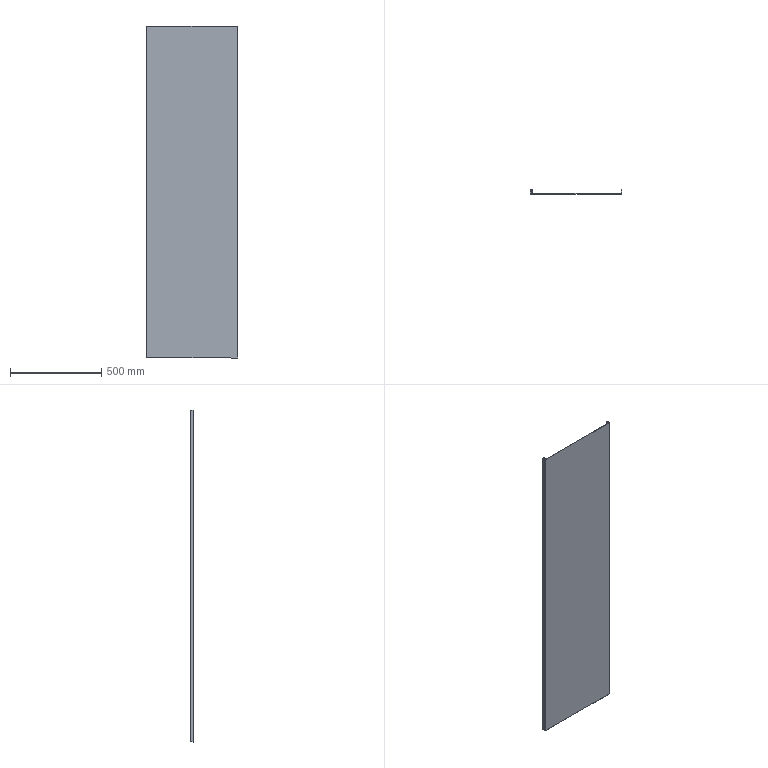Component | SolidWorks | SidePlate-1 | 1 solid | 38 faces | box 500 x 20 x 1820 mm | volume 1504835 mm3 | plane 30 | cylinder 8 | commonest cylinder face diameters 5 x2 2 x2 4.473 x2 1.473 x2
STEP:
#1=COLOUR_RGB('',0.7922,0.8196,0.9333);
#2=FILL_AREA_STYLE_COLOUR('',#1);
#3=FILL_AREA_STYLE('',(#2));
#4=SURFACE_STYLE_FILL_AREA(#3);
#5=SURFACE_SIDE_STYLE('',(#4));
#6=SURFACE_STYLE_USAGE(.BOTH.,#5);
#7=PRESENTATION_STYLE_ASSIGNMENT((#6));
#8=CARTESIAN_POINT('',(0.2466,-9.272,66.594));
#9=VERTEX_POINT('',#8);
#10=CARTESIAN_POINT('',(0.029,-9.272,66.594));
#11=VERTEX_POINT('',#10);
#12=CARTESIAN_POINT('',(9.783,-9.272,66.594));
#13=DIRECTION('',(-1.,-0.,0.));
#14=VECTOR('',#13,39.37);
#15=LINE('',#12,#14);
#16=EDGE_CURVE('',#9,#11,#15,.T.);
#17=ORIENTED_EDGE('',*,*,#16,.F.);
#18=CARTESIAN_POINT('',(0.2466,-9.213,66.594));
#19=VERTEX_POINT('',#18);
#20=CARTESIAN_POINT('',(0.2466,-9.272,66.594));
#21=DIRECTION('',(0.,1.,0.));
#22=VECTOR('',#21,39.37);
#23=LINE('',#20,#22);
#24=EDGE_CURVE('',#9,#19,#23,.T.);
#25=ORIENTED_EDGE('',*,*,#24,.T.);
#26=CARTESIAN_POINT('',(0.029,-9.213,66.594));
#27=VERTEX_POINT('',#26);
#28=CARTESIAN_POINT('',(0.,-9.213,66.594));
#29=DIRECTION('',(-1.,-0.,0.));
#30=VECTOR('',#29,39.37);
#31=LINE('',#28,#30);
#32=EDGE_CURVE('',#19,#27,#31,.T.);
#33=ORIENTED_EDGE('',*,*,#32,.T.);
#34=CARTESIAN_POINT('',(0.029,-9.272,66.594));
#35=DIRECTION('',(-0.,1.,0.));
#36=VECTOR('',#35,39.37);
#37=LINE('',#34,#36);
#38=EDGE_CURVE('',#11,#27,#37,.T.);
#39=ORIENTED_EDGE('',*,*,#38,.F.);
#40=EDGE_LOOP('',(#17,#25,#33,#39));
#41=FACE_OUTER_BOUND('',#40,.T.);
#42=CARTESIAN_POINT('',(0.,-9.213,66.594));
#43=DIRECTION('',(0.,-0.,1.));
#44=DIRECTION('',(-1.,0.,0.));
#45=AXIS2_PLACEMENT_3D('',#42,#43,#44);
#46=PLANE('',#45);
#47=ADVANCED_FACE('',(#41),#46,.T.);
#48=ORIENTED_EDGE('',*,*,#32,.F.);
#49=CARTESIAN_POINT('',(0.2466,-9.213,-5.059));
#50=VERTEX_POINT('',#49);
#51=CARTESIAN_POINT('',(0.2466,-9.213,66.594));
#52=DIRECTION('',(-0.,0.,-1.));
#53=VECTOR('',#52,39.37);
#54=LINE('',#51,#53);
#55=EDGE_CURVE('',#19,#50,#54,.T.);
#56=ORIENTED_EDGE('',*,*,#55,.T.);
#57=CARTESIAN_POINT('',(0.029,-9.213,-5.059));
#58=VERTEX_POINT('',#57);
#59=CARTESIAN_POINT('',(0.3346,-9.213,-5.059));
#60=DIRECTION('',(1.,0.,-0.));
#61=VECTOR('',#60,39.37);
#62=LINE('',#59,#61);
#63=EDGE_CURVE('',#58,#50,#62,.T.);
#64=ORIENTED_EDGE('',*,*,#63,.F.);
#65=CARTESIAN_POINT('',(0.029,-9.213,30.768));
#66=DIRECTION('',(0.,-0.,1.));
#67=VECTOR('',#66,39.37);
#68=LINE('',#65,#67);
#69=EDGE_CURVE('',#58,#27,#68,.T.);
#70=ORIENTED_EDGE('',*,*,#69,.T.);
#71=EDGE_LOOP('',(#48,#56,#64,#70));
#72=FACE_OUTER_BOUND('',#71,.T.);
#73=CARTESIAN_POINT('',(9.783,-9.213,30.768));
#74=DIRECTION('',(-0.,1.,0.));
#75=DIRECTION('',(1.,0.,-0.));
#76=AXIS2_PLACEMENT_3D('',#73,#74,#75);
#77=PLANE('',#76);
#78=ADVANCED_FACE('',(#72),#77,.T.);
#79=CARTESIAN_POINT('',(0.2466,-9.272,-5.059));
#80=VERTEX_POINT('',#79);
#81=CARTESIAN_POINT('',(0.2466,-9.272,66.594));
#82=DIRECTION('',(-0.,0.,-1.));
#83=VECTOR('',#82,39.37);
#84=LINE('',#81,#83);
#85=EDGE_CURVE('',#9,#80,#84,.T.);
#86=ORIENTED_EDGE('',*,*,#85,.F.);
#87=ORIENTED_EDGE('',*,*,#16,.T.);
#88=CARTESIAN_POINT('',(0.029,-9.272,-5.059));
#89=VERTEX_POINT('',#88);
#90=CARTESIAN_POINT('',(0.029,-9.272,-5.059));
#91=DIRECTION('',(0.,-0.,1.));
#92=VECTOR('',#91,39.37);
#93=LINE('',#90,#92);
#94=EDGE_CURVE('',#89,#11,#93,.T.);
#95=ORIENTED_EDGE('',*,*,#94,.F.);
#96=CARTESIAN_POINT('',(9.783,-9.272,-5.059));
#97=DIRECTION('',(1.,0.,-0.));
#98=VECTOR('',#97,39.37);
#99=LINE('',#96,#98);
#100=EDGE_CURVE('',#89,#80,#99,.T.);
#101=ORIENTED_EDGE('',*,*,#100,.T.);
#102=EDGE_LOOP('',(#86,#87,#95,#101));
#103=FACE_OUTER_BOUND('',#102,.T.);
#104=CARTESIAN_POINT('',(9.783,-9.272,30.768));
#105=DIRECTION('',(-0.,1.,0.));
#106=DIRECTION('',(1.,0.,-0.));
#107=AXIS2_PLACEMENT_3D('',#104,#105,#106);
#108=PLANE('',#107);
#109=ADVANCED_FACE('',(#103),#108,.F.);
#110=CARTESIAN_POINT('',(0.,-9.301,66.594));
#111=VERTEX_POINT('',#110);
#112=CARTESIAN_POINT('',(0.,-9.902,66.594));
#113=VERTEX_POINT('',#112);
#114=CARTESIAN_POINT('',(0.,-10.,66.594));
#115=DIRECTION('',(0.,-1.,-0.));
#116=VECTOR('',#115,39.37);
#117=LINE('',#114,#116);
#118=EDGE_CURVE('',#111,#113,#117,.T.);
#119=ORIENTED_EDGE('',*,*,#118,.F.);
#120=CARTESIAN_POINT('',(-0.05906,-9.301,66.594));
#121=VERTEX_POINT('',#120);
#122=CARTESIAN_POINT('',(0.,-9.301,66.594));
#123=DIRECTION('',(-1.,-0.,0.));
#124=VECTOR('',#123,39.37);
#125=LINE('',#122,#124);
#126=EDGE_CURVE('',#111,#121,#125,.T.);
#127=ORIENTED_EDGE('',*,*,#126,.T.);
#128=CARTESIAN_POINT('',(-0.05906,-9.902,66.594));
#129=VERTEX_POINT('',#128);
#130=CARTESIAN_POINT('',(-0.05906,-9.213,66.594));
#131=DIRECTION('',(0.,-1.,-0.));
#132=VECTOR('',#131,39.37);
#133=LINE('',#130,#132);
#134=EDGE_CURVE('',#121,#129,#133,.T.);
#135=ORIENTED_EDGE('',*,*,#134,.T.);
#136=CARTESIAN_POINT('',(0.,-9.902,66.594));
#137=DIRECTION('',(-1.,0.,0.));
#138=VECTOR('',#137,39.37);
#139=LINE('',#136,#138);
#140=EDGE_CURVE('',#113,#129,#139,.T.);
#141=ORIENTED_EDGE('',*,*,#140,.F.);
#142=EDGE_LOOP('',(#119,#127,#135,#141));
#143=FACE_OUTER_BOUND('',#142,.T.);
#144=CARTESIAN_POINT('',(-0.05906,-9.213,66.594));
#145=DIRECTION('',(0.,-0.,1.));
#146=DIRECTION('',(-1.,0.,0.));
#147=AXIS2_PLACEMENT_3D('',#144,#145,#146);
#148=PLANE('',#147);
#149=ADVANCED_FACE('',(#143),#148,.T.);
#150=CARTESIAN_POINT('',(-0.05906,-9.301,-5.059));
#151=VERTEX_POINT('',#150);
#152=CARTESIAN_POINT('',(-0.05906,-9.301,66.594));
#153=DIRECTION('',(-0.,0.,-1.));
#154=VECTOR('',#153,39.37);
#155=LINE('',#152,#154);
#156=EDGE_CURVE('',#121,#151,#155,.T.);
#157=ORIENTED_EDGE('',*,*,#156,.T.);
#158=CARTESIAN_POINT('',(-0.05906,-9.902,-5.059));
#159=VERTEX_POINT('',#158);
#160=CARTESIAN_POINT('',(-0.05906,-9.941,-5.059));
#161=DIRECTION('',(-0.,1.,0.));
#162=VECTOR('',#161,39.37);
#163=LINE('',#160,#162);
#164=EDGE_CURVE('',#159,#151,#163,.T.);
#165=ORIENTED_EDGE('',*,*,#164,.F.);
#166=CARTESIAN_POINT('',(-0.05906,-9.902,-5.059));
#167=DIRECTION('',(-0.,0.,-1.));
#168=VECTOR('',#167,39.37);
#169=LINE('',#166,#168);
#170=EDGE_CURVE('',#129,#159,#169,.T.);
#171=ORIENTED_EDGE('',*,*,#170,.F.);
#172=ORIENTED_EDGE('',*,*,#134,.F.);
#173=EDGE_LOOP('',(#157,#165,#171,#172));
#174=FACE_OUTER_BOUND('',#173,.T.);
#175=CARTESIAN_POINT('',(-0.05906,-10.,30.768));
#176=DIRECTION('',(1.,0.,-0.));
#177=DIRECTION('',(0.,-1.,-0.));
#178=AXIS2_PLACEMENT_3D('',#175,#176,#177);
#179=PLANE('',#178);
#180=ADVANCED_FACE('',(#174),#179,.F.);
#181=CARTESIAN_POINT('',(0.,-9.902,-5.059));
#182=VERTEX_POINT('',#181);
#183=CARTESIAN_POINT('',(0.,-9.301,-5.059));
#184=VERTEX_POINT('',#183);
#185=CARTESIAN_POINT('',(0.,-10.,-5.059));
#186=DIRECTION('',(-0.,1.,0.));
#187=VECTOR('',#186,39.37);
#188=LINE('',#185,#187);
#189=EDGE_CURVE('',#182,#184,#188,.T.);
#190=ORIENTED_EDGE('',*,*,#189,.T.);
#191=CARTESIAN_POINT('',(0.,-9.301,66.594));
#192=DIRECTION('',(-0.,0.,-1.));
#193=VECTOR('',#192,39.37);
#194=LINE('',#191,#193);
#195=EDGE_CURVE('',#111,#184,#194,.T.);
#196=ORIENTED_EDGE('',*,*,#195,.F.);
#197=ORIENTED_EDGE('',*,*,#118,.T.);
#198=CARTESIAN_POINT('',(0.,-9.902,-5.059));
#199=DIRECTION('',(0.,-0.,1.));
#200=VECTOR('',#199,39.37);
#201=LINE('',#198,#200);
#202=EDGE_CURVE('',#182,#113,#201,.T.);
#203=ORIENTED_EDGE('',*,*,#202,.F.);
#204=EDGE_LOOP('',(#190,#196,#197,#203));
#205=FACE_OUTER_BOUND('',#204,.T.);
#206=CARTESIAN_POINT('',(0.,-10.,30.768));
#207=DIRECTION('',(1.,0.,-0.));
#208=DIRECTION('',(0.,-1.,-0.));
#209=AXIS2_PLACEMENT_3D('',#206,#207,#208);
#210=PLANE('',#209);
#211=ADVANCED_FACE('',(#205),#210,.T.);
#212=CARTESIAN_POINT('',(0.03937,-9.941,66.594));
#213=VERTEX_POINT('',#212);
#214=CARTESIAN_POINT('',(0.03937,-9.941,-5.059));
#215=VERTEX_POINT('',#214);
#216=CARTESIAN_POINT('',(0.03937,-9.941,66.594));
#217=DIRECTION('',(-0.,0.,-1.));
#218=VECTOR('',#217,39.37);
#219=LINE('',#216,#218);
#220=EDGE_CURVE('',#213,#215,#219,.T.);
#221=ORIENTED_EDGE('',*,*,#220,.F.);
#222=CARTESIAN_POINT('',(19.528,-9.941,66.594));
#223=VERTEX_POINT('',#222);
#224=CARTESIAN_POINT('',(19.626,-9.941,66.594));
#225=DIRECTION('',(-1.,0.,0.));
#226=VECTOR('',#225,39.37);
#227=LINE('',#224,#226);
#228=EDGE_CURVE('',#223,#213,#227,.T.);
#229=ORIENTED_EDGE('',*,*,#228,.F.);
#230=CARTESIAN_POINT('',(19.528,-9.941,-5.059));
#231=VERTEX_POINT('',#230);
#232=CARTESIAN_POINT('',(19.528,-9.941,-5.059));
#233=DIRECTION('',(0.,-0.,1.));
#234=VECTOR('',#233,39.37);
#235=LINE('',#232,#234);
#236=EDGE_CURVE('',#231,#223,#235,.T.);
#237=ORIENTED_EDGE('',*,*,#236,.F.);
#238=CARTESIAN_POINT('',(19.626,-9.941,-5.059));
#239=DIRECTION('',(1.,-0.,-0.));
#240=VECTOR('',#239,39.37);
#241=LINE('',#238,#240);
#242=EDGE_CURVE('',#215,#231,#241,.T.);
#243=ORIENTED_EDGE('',*,*,#242,.F.);
#244=EDGE_LOOP('',(#221,#229,#237,#243));
#245=FACE_OUTER_BOUND('',#244,.T.);
#246=CARTESIAN_POINT('',(9.783,-9.941,30.768));
#247=DIRECTION('',(-0.,-1.,-0.));
#248=DIRECTION('',(-1.,0.,0.));
#249=AXIS2_PLACEMENT_3D('',#246,#247,#248);
#250=PLANE('',#249);
#251=ADVANCED_FACE('',(#245),#250,.F.);
#252=CARTESIAN_POINT('',(19.528,-10.,66.594));
#253=VERTEX_POINT('',#252);
#254=CARTESIAN_POINT('',(0.03937,-10.,66.594));
#255=VERTEX_POINT('',#254);
#256=CARTESIAN_POINT('',(19.626,-10.,66.594));
#257=DIRECTION('',(-1.,0.,0.));
#258=VECTOR('',#257,39.37);
#259=LINE('',#256,#258);
#260=EDGE_CURVE('',#253,#255,#259,.T.);
#261=ORIENTED_EDGE('',*,*,#260,.T.);
#262=CARTESIAN_POINT('',(0.03937,-10.,-5.059));
#263=VERTEX_POINT('',#262);
#264=CARTESIAN_POINT('',(0.03937,-10.,66.594));
#265=DIRECTION('',(-0.,0.,-1.));
#266=VECTOR('',#265,39.37);
#267=LINE('',#264,#266);
#268=EDGE_CURVE('',#255,#263,#267,.T.);
#269=ORIENTED_EDGE('',*,*,#268,.T.);
#270=CARTESIAN_POINT('',(19.528,-10.,-5.059));
#271=VERTEX_POINT('',#270);
#272=CARTESIAN_POINT('',(19.626,-10.,-5.059));
#273=DIRECTION('',(1.,-0.,-0.));
#274=VECTOR('',#273,39.37);
#275=LINE('',#272,#274);
#276=EDGE_CURVE('',#263,#271,#275,.T.);
#277=ORIENTED_EDGE('',*,*,#276,.T.);
#278=CARTESIAN_POINT('',(19.528,-10.,-5.059));
#279=DIRECTION('',(0.,-0.,1.));
#280=VECTOR('',#279,39.37);
#281=LINE('',#278,#280);
#282=EDGE_CURVE('',#271,#253,#281,.T.);
#283=ORIENTED_EDGE('',*,*,#282,.T.);
#284=EDGE_LOOP('',(#261,#269,#277,#283));
#285=FACE_OUTER_BOUND('',#284,.T.);
#286=CARTESIAN_POINT('',(9.783,-10.,30.768));
#287=DIRECTION('',(-0.,-1.,-0.));
#288=DIRECTION('',(-1.,0.,0.));
#289=AXIS2_PLACEMENT_3D('',#286,#287,#288);
#290=PLANE('',#289);
#291=ADVANCED_FACE('',(#285),#290,.T.);
#292=ORIENTED_EDGE('',*,*,#228,.T.);
#293=CARTESIAN_POINT('',(0.03937,-9.941,66.594));
#294=DIRECTION('',(-0.,-1.,-0.));
#295=VECTOR('',#294,39.37);
#296=LINE('',#293,#295);
#297=EDGE_CURVE('',#213,#255,#296,.T.);
#298=ORIENTED_EDGE('',*,*,#297,.T.);
#299=ORIENTED_EDGE('',*,*,#260,.F.);
#300=CARTESIAN_POINT('',(19.528,-9.941,66.594));
#301=DIRECTION('',(-0.,-1.,-0.));
#302=VECTOR('',#301,39.37);
#303=LINE('',#300,#302);
#304=EDGE_CURVE('',#223,#253,#303,.T.);
#305=ORIENTED_EDGE('',*,*,#304,.F.);
#306=EDGE_LOOP('',(#292,#298,#299,#305));
#307=FACE_OUTER_BOUND('',#306,.T.);
#308=CARTESIAN_POINT('',(19.626,-9.941,66.594));
#309=DIRECTION('',(0.,-0.,1.));
#310=DIRECTION('',(-1.,0.,0.));
#311=AXIS2_PLACEMENT_3D('',#308,#309,#310);
#312=PLANE('',#311);
#313=ADVANCED_FACE('',(#307),#312,.T.);
#314=CARTESIAN_POINT('',(0.03937,-9.941,-5.059));
#315=DIRECTION('',(-0.,-1.,-0.));
#316=VECTOR('',#315,39.37);
#317=LINE('',#314,#316);
#318=EDGE_CURVE('',#215,#263,#317,.T.);
#319=ORIENTED_EDGE('',*,*,#318,.F.);
#320=ORIENTED_EDGE('',*,*,#242,.T.);
#321=CARTESIAN_POINT('',(19.528,-9.941,-5.059));
#322=DIRECTION('',(-0.,-1.,-0.));
#323=VECTOR('',#322,39.37);
#324=LINE('',#321,#323);
#325=EDGE_CURVE('',#231,#271,#324,.T.);
#326=ORIENTED_EDGE('',*,*,#325,.T.);
#327=ORIENTED_EDGE('',*,*,#276,.F.);
#328=EDGE_LOOP('',(#319,#320,#326,#327));
#329=FACE_OUTER_BOUND('',#328,.T.);
#330=CARTESIAN_POINT('',(19.626,-9.941,-5.059));
#331=DIRECTION('',(-0.,0.,-1.));
#332=DIRECTION('',(1.,-0.,-0.));
#333=AXIS2_PLACEMENT_3D('',#330,#331,#332);
#334=PLANE('',#333);
#335=ADVANCED_FACE('',(#329),#334,.T.);
#336=CARTESIAN_POINT('',(19.567,-9.902,66.594));
#337=VERTEX_POINT('',#336);
#338=CARTESIAN_POINT('',(19.626,-9.902,66.594));
#339=VERTEX_POINT('',#338);
#340=CARTESIAN_POINT('',(19.626,-9.902,66.594));
#341=DIRECTION('',(1.,-0.,-0.));
#342=VECTOR('',#341,39.37);
#343=LINE('',#340,#342);
#344=EDGE_CURVE('',#337,#339,#343,.T.);
#345=ORIENTED_EDGE('',*,*,#344,.F.);
#346=CARTESIAN_POINT('',(19.528,-9.902,66.594));
#347=DIRECTION('',(0.,-0.,1.));
#348=DIRECTION('',(1.,0.,0.));
#349=AXIS2_PLACEMENT_3D('',#346,#347,#348);
#350=CIRCLE('',#349,0.03937);
#351=EDGE_CURVE('',#223,#337,#350,.T.);
#352=ORIENTED_EDGE('',*,*,#351,.F.);
#353=ORIENTED_EDGE('',*,*,#304,.T.);
#354=CARTESIAN_POINT('',(19.528,-9.902,66.594));
#355=DIRECTION('',(0.,-0.,1.));
#356=DIRECTION('',(1.,0.,0.));
#357=AXIS2_PLACEMENT_3D('',#354,#355,#356);
#358=CIRCLE('',#357,0.09843);
#359=EDGE_CURVE('',#253,#339,#358,.T.);
#360=ORIENTED_EDGE('',*,*,#359,.T.);
#361=EDGE_LOOP('',(#345,#352,#353,#360));
#362=FACE_OUTER_BOUND('',#361,.T.);
#363=CARTESIAN_POINT('',(19.528,-9.902,66.594));
#364=DIRECTION('',(0.,-0.,1.));
#365=DIRECTION('',(-1.,0.,0.));
#366=AXIS2_PLACEMENT_3D('',#363,#364,#365);
#367=PLANE('',#366);
#368=ADVANCED_FACE('',(#362),#367,.T.);
#369=CARTESIAN_POINT('',(19.567,-9.902,-5.059));
#370=VERTEX_POINT('',#369);
#371=CARTESIAN_POINT('',(19.528,-9.902,-5.059));
#372=DIRECTION('',(-0.,0.,-1.));
#373=DIRECTION('',(1.,0.,0.));
#374=AXIS2_PLACEMENT_3D('',#371,#372,#373);
#375=CIRCLE('',#374,0.03937);
#376=EDGE_CURVE('',#370,#231,#375,.T.);
#377=ORIENTED_EDGE('',*,*,#376,.F.);
#378=CARTESIAN_POINT('',(19.626,-9.902,-5.059));
#379=VERTEX_POINT('',#378);
#380=CARTESIAN_POINT('',(19.567,-9.902,-5.059));
#381=DIRECTION('',(1.,-0.,-0.));
#382=VECTOR('',#381,39.37);
#383=LINE('',#380,#382);
#384=EDGE_CURVE('',#370,#379,#383,.T.);
#385=ORIENTED_EDGE('',*,*,#384,.T.);
#386=CARTESIAN_POINT('',(19.528,-9.902,-5.059));
#387=DIRECTION('',(-0.,0.,-1.));
#388=DIRECTION('',(1.,0.,0.));
#389=AXIS2_PLACEMENT_3D('',#386,#387,#388);
#390=CIRCLE('',#389,0.09843);
#391=EDGE_CURVE('',#379,#271,#390,.T.);
#392=ORIENTED_EDGE('',*,*,#391,.T.);
#393=ORIENTED_EDGE('',*,*,#325,.F.);
#394=EDGE_LOOP('',(#377,#385,#392,#393));
#395=FACE_OUTER_BOUND('',#394,.T.);
#396=CARTESIAN_POINT('',(19.528,-9.902,-5.059));
#397=DIRECTION('',(0.,-0.,1.));
#398=DIRECTION('',(-1.,0.,0.));
#399=AXIS2_PLACEMENT_3D('',#396,#397,#398);
#400=PLANE('',#399);
#401=ADVANCED_FACE('',(#395),#400,.F.);
#402=ORIENTED_EDGE('',*,*,#282,.F.);
#403=ORIENTED_EDGE('',*,*,#391,.F.);
#404=CARTESIAN_POINT('',(19.626,-9.902,30.768));
#405=DIRECTION('',(-0.,0.,-1.));
#406=VECTOR('',#405,39.37);
#407=LINE('',#404,#406);
#408=EDGE_CURVE('',#339,#379,#407,.T.);
#409=ORIENTED_EDGE('',*,*,#408,.F.);
#410=ORIENTED_EDGE('',*,*,#359,.F.);
#411=EDGE_LOOP('',(#402,#403,#409,#410));
#412=FACE_OUTER_BOUND('',#411,.T.);
#413=CARTESIAN_POINT('',(19.528,-9.902,-5.059));
#414=DIRECTION('',(-0.,0.,-1.));
#415=DIRECTION('',(1.,0.,0.));
#416=AXIS2_PLACEMENT_3D('',#413,#414,#415);
#417=CYLINDRICAL_SURFACE('',#416,0.09843);
#418=ADVANCED_FACE('',(#412),#417,.T.);
#419=ORIENTED_EDGE('',*,*,#236,.T.);
#420=ORIENTED_EDGE('',*,*,#351,.T.);
#421=CARTESIAN_POINT('',(19.567,-9.902,66.594));
#422=DIRECTION('',(-0.,0.,-1.));
#423=VECTOR('',#422,39.37);
#424=LINE('',#421,#423);
#425=EDGE_CURVE('',#337,#370,#424,.T.);
#426=ORIENTED_EDGE('',*,*,#425,.T.);
#427=ORIENTED_EDGE('',*,*,#376,.T.);
#428=EDGE_LOOP('',(#419,#420,#426,#427));
#429=FACE_OUTER_BOUND('',#428,.T.);
#430=CARTESIAN_POINT('',(19.528,-9.902,-5.059));
#431=DIRECTION('',(-0.,0.,-1.));
#432=DIRECTION('',(1.,0.,0.));
#433=AXIS2_PLACEMENT_3D('',#430,#431,#432);
#434=CYLINDRICAL_SURFACE('',#433,0.03937);
#435=ADVANCED_FACE('',(#429),#434,.F.);
#436=CARTESIAN_POINT('',(19.626,-9.213,-5.059));
#437=VERTEX_POINT('',#436);
#438=CARTESIAN_POINT('',(19.626,-9.941,-5.059));
#439=DIRECTION('',(-0.,-1.,-0.));
#440=VECTOR('',#439,39.37);
#441=LINE('',#438,#440);
#442=EDGE_CURVE('',#437,#379,#441,.T.);
#443=ORIENTED_EDGE('',*,*,#442,.T.);
#444=ORIENTED_EDGE('',*,*,#384,.F.);
#445=CARTESIAN_POINT('',(19.567,-9.213,-5.059));
#446=VERTEX_POINT('',#445);
#447=CARTESIAN_POINT('',(19.567,-10.,-5.059));
#448=DIRECTION('',(-0.,-1.,-0.));
#449=VECTOR('',#448,39.37);
#450=LINE('',#447,#449);
#451=EDGE_CURVE('',#446,#370,#450,.T.);
#452=ORIENTED_EDGE('',*,*,#451,.F.);
#453=CARTESIAN_POINT('',(19.626,-9.213,-5.059));
#454=DIRECTION('',(-1.,0.,0.));
#455=VECTOR('',#454,39.37);
#456=LINE('',#453,#455);
#457=EDGE_CURVE('',#437,#446,#456,.T.);
#458=ORIENTED_EDGE('',*,*,#457,.F.);
#459=EDGE_LOOP('',(#443,#444,#452,#458));
#460=FACE_OUTER_BOUND('',#459,.T.);
#461=CARTESIAN_POINT('',(19.626,-9.941,-5.059));
#462=DIRECTION('',(-0.,0.,-1.));
#463=DIRECTION('',(-0.,-1.,-0.));
#464=AXIS2_PLACEMENT_3D('',#461,#462,#463);
#465=PLANE('',#464);
#466=ADVANCED_FACE('',(#460),#465,.T.);
#467=CARTESIAN_POINT('',(19.567,-9.213,66.594));
#468=VERTEX_POINT('',#467);
#469=CARTESIAN_POINT('',(19.567,-10.,66.594));
#470=DIRECTION('',(0.,1.,0.));
#471=VECTOR('',#470,39.37);
#472=LINE('',#469,#471);
#473=EDGE_CURVE('',#337,#468,#472,.T.);
#474=ORIENTED_EDGE('',*,*,#473,.F.);
#475=ORIENTED_EDGE('',*,*,#344,.T.);
#476=CARTESIAN_POINT('',(19.626,-9.213,66.594));
#477=VERTEX_POINT('',#476);
#478=CARTESIAN_POINT('',(19.626,-9.213,66.594));
#479=DIRECTION('',(0.,1.,0.));
#480=VECTOR('',#479,39.37);
#481=LINE('',#478,#480);
#482=EDGE_CURVE('',#339,#477,#481,.T.);
#483=ORIENTED_EDGE('',*,*,#482,.T.);
#484=CARTESIAN_POINT('',(19.626,-9.213,66.594));
#485=DIRECTION('',(-1.,0.,0.));
#486=VECTOR('',#485,39.37);
#487=LINE('',#484,#486);
#488=EDGE_CURVE('',#477,#468,#487,.T.);
#489=ORIENTED_EDGE('',*,*,#488,.T.);
#490=EDGE_LOOP('',(#474,#475,#483,#489));
#491=FACE_OUTER_BOUND('',#490,.T.);
#492=CARTESIAN_POINT('',(19.626,-9.213,66.594));
#493=DIRECTION('',(0.,-0.,1.));
#494=DIRECTION('',(0.,1.,0.));
#495=AXIS2_PLACEMENT_3D('',#492,#493,#494);
#496=PLANE('',#495);
#497=ADVANCED_FACE('',(#491),#496,.T.);
#498=ORIENTED_EDGE('',*,*,#482,.F.);
#499=ORIENTED_EDGE('',*,*,#408,.T.);
#500=ORIENTED_EDGE('',*,*,#442,.F.);
#501=CARTESIAN_POINT('',(19.626,-9.213,-5.059));
#502=DIRECTION('',(-0.,0.,-1.));
#503=VECTOR('',#502,39.37);
#504=LINE('',#501,#503);
#505=EDGE_CURVE('',#477,#437,#504,.T.);
#506=ORIENTED_EDGE('',*,*,#505,.F.);
#507=EDGE_LOOP('',(#498,#499,#500,#506));
#508=FACE_OUTER_BOUND('',#507,.T.);
#509=CARTESIAN_POINT('',(19.626,-10.,30.768));
#510=DIRECTION('',(1.,-0.,-0.));
#511=DIRECTION('',(-0.,-1.,-0.));
#512=AXIS2_PLACEMENT_3D('',#509,#510,#511);
#513=PLANE('',#512);
#514=ADVANCED_FACE('',(#508),#513,.T.);
#515=ORIENTED_EDGE('',*,*,#425,.F.);
#516=ORIENTED_EDGE('',*,*,#473,.T.);
#517=CARTESIAN_POINT('',(19.567,-9.213,30.768));
#518=DIRECTION('',(-0.,0.,-1.));
#519=VECTOR('',#518,39.37);
#520=LINE('',#517,#519);
#521=EDGE_CURVE('',#468,#446,#520,.T.);
#522=ORIENTED_EDGE('',*,*,#521,.T.);
#523=ORIENTED_EDGE('',*,*,#451,.T.);
#524=EDGE_LOOP('',(#515,#516,#522,#523));
#525=FACE_OUTER_BOUND('',#524,.T.);
#526=CARTESIAN_POINT('',(19.567,-10.,30.768));
#527=DIRECTION('',(1.,-0.,-0.));
#528=DIRECTION('',(-0.,-1.,-0.));
#529=AXIS2_PLACEMENT_3D('',#526,#527,#528);
#530=PLANE('',#529);
#531=ADVANCED_FACE('',(#525),#530,.F.);
#532=ORIENTED_EDGE('',*,*,#521,.F.);
#533=ORIENTED_EDGE('',*,*,#488,.F.);
#534=ORIENTED_EDGE('',*,*,#505,.T.);
#535=ORIENTED_EDGE('',*,*,#457,.T.);
#536=EDGE_LOOP('',(#532,#533,#534,#535));
#537=FACE_OUTER_BOUND('',#536,.T.);
#538=CARTESIAN_POINT('',(19.626,-9.213,-5.059));
#539=DIRECTION('',(0.,1.,0.));
#540=DIRECTION('',(1.,-0.,-0.));
#541=AXIS2_PLACEMENT_3D('',#538,#539,#540);
#542=PLANE('',#541);
#543=ADVANCED_FACE('',(#537),#542,.T.);
#544=CARTESIAN_POINT('',(-0.05906,-9.902,-5.059));
#545=DIRECTION('',(-1.,0.,0.));
#546=VECTOR('',#545,39.37);
#547=LINE('',#544,#546);
#548=EDGE_CURVE('',#182,#159,#547,.T.);
#549=ORIENTED_EDGE('',*,*,#548,.F.);
#550=CARTESIAN_POINT('',(0.03937,-9.902,-5.059));
#551=DIRECTION('',(-0.,0.,-1.));
#552=DIRECTION('',(-1.,0.,0.));
#553=AXIS2_PLACEMENT_3D('',#550,#551,#552);
#554=CIRCLE('',#553,0.03937);
#555=EDGE_CURVE('',#215,#182,#554,.T.);
#556=ORIENTED_EDGE('',*,*,#555,.F.);
#557=ORIENTED_EDGE('',*,*,#318,.T.);
#558=CARTESIAN_POINT('',(0.03937,-9.902,-5.059));
#559=DIRECTION('',(-0.,0.,-1.));
#560=DIRECTION('',(-1.,0.,0.));
#561=AXIS2_PLACEMENT_3D('',#558,#559,#560);
#562=CIRCLE('',#561,0.09843);
#563=EDGE_CURVE('',#263,#159,#562,.T.);
#564=ORIENTED_EDGE('',*,*,#563,.T.);
#565=EDGE_LOOP('',(#549,#556,#557,#564));
#566=FACE_OUTER_BOUND('',#565,.T.);
#567=CARTESIAN_POINT('',(0.03937,-9.902,-5.059));
#568=DIRECTION('',(-0.,0.,-1.));
#569=DIRECTION('',(1.,-0.,-0.));
#570=AXIS2_PLACEMENT_3D('',#567,#568,#569);
#571=PLANE('',#570);
#572=ADVANCED_FACE('',(#566),#571,.T.);
#573=CARTESIAN_POINT('',(0.03937,-9.902,66.594));
#574=DIRECTION('',(0.,-0.,1.));
#575=DIRECTION('',(-1.,0.,0.));
#576=AXIS2_PLACEMENT_3D('',#573,#574,#575);
#577=CIRCLE('',#576,0.03937);
#578=EDGE_CURVE('',#113,#213,#577,.T.);
#579=ORIENTED_EDGE('',*,*,#578,.F.);
#580=ORIENTED_EDGE('',*,*,#140,.T.);
#581=CARTESIAN_POINT('',(0.03937,-9.902,66.594));
#582=DIRECTION('',(0.,-0.,1.));
#583=DIRECTION('',(-1.,0.,0.));
#584=AXIS2_PLACEMENT_3D('',#581,#582,#583);
#585=CIRCLE('',#584,0.09843);
#586=EDGE_CURVE('',#129,#255,#585,.T.);
#587=ORIENTED_EDGE('',*,*,#586,.T.);
#588=ORIENTED_EDGE('',*,*,#297,.F.);
#589=EDGE_LOOP('',(#579,#580,#587,#588));
#590=FACE_OUTER_BOUND('',#589,.T.);
#591=CARTESIAN_POINT('',(0.03937,-9.902,66.594));
#592=DIRECTION('',(-0.,0.,-1.));
#593=DIRECTION('',(1.,-0.,-0.));
#594=AXIS2_PLACEMENT_3D('',#591,#592,#593);
#595=PLANE('',#594);
#596=ADVANCED_FACE('',(#590),#595,.F.);
#597=ORIENTED_EDGE('',*,*,#268,.F.);
#598=ORIENTED_EDGE('',*,*,#586,.F.);
#599=ORIENTED_EDGE('',*,*,#170,.T.);
#600=ORIENTED_EDGE('',*,*,#563,.F.);
#601=EDGE_LOOP('',(#597,#598,#599,#600));
#602=FACE_OUTER_BOUND('',#601,.T.);
#603=CARTESIAN_POINT('',(0.03937,-9.902,66.594));
#604=DIRECTION('',(0.,-0.,1.));
#605=DIRECTION('',(-1.,0.,0.));
#606=AXIS2_PLACEMENT_3D('',#603,#604,#605);
#607=CYLINDRICAL_SURFACE('',#606,0.09843);
#608=ADVANCED_FACE('',(#602),#607,.T.);
#609=ORIENTED_EDGE('',*,*,#220,.T.);
#610=ORIENTED_EDGE('',*,*,#555,.T.);
#611=ORIENTED_EDGE('',*,*,#202,.T.);
#612=ORIENTED_EDGE('',*,*,#578,.T.);
#613=EDGE_LOOP('',(#609,#610,#611,#612));
#614=FACE_OUTER_BOUND('',#613,.T.);
#615=CARTESIAN_POINT('',(0.03937,-9.902,66.594));
#616=DIRECTION('',(0.,-0.,1.));
#617=DIRECTION('',(-1.,0.,0.));
#618=AXIS2_PLACEMENT_3D('',#615,#616,#617);
#619=CYLINDRICAL_SURFACE('',#618,0.03937);
#620=ADVANCED_FACE('',(#614),#619,.F.);
#621=CARTESIAN_POINT('',(0.,-9.301,-5.059));
#622=DIRECTION('',(-1.,-0.,0.));
#623=VECTOR('',#622,39.37);
#624=LINE('',#621,#623);
#625=EDGE_CURVE('',#184,#151,#624,.T.);
#626=ORIENTED_EDGE('',*,*,#625,.F.);
#627=ORIENTED_EDGE('',*,*,#189,.F.);
#628=ORIENTED_EDGE('',*,*,#548,.T.);
#629=ORIENTED_EDGE('',*,*,#164,.T.);
#630=EDGE_LOOP('',(#626,#627,#628,#629));
#631=FACE_OUTER_BOUND('',#630,.T.);
#632=CARTESIAN_POINT('',(-0.05906,-9.941,-5.059));
#633=DIRECTION('',(-0.,0.,-1.));
#634=DIRECTION('',(1.,-0.,-0.));
#635=AXIS2_PLACEMENT_3D('',#632,#633,#634);
#636=PLANE('',#635);
#637=ADVANCED_FACE('',(#631),#636,.T.);
#638=CARTESIAN_POINT('',(0.029,-9.213,-5.059));
#639=DIRECTION('',(-0.,1.,0.));
#640=VECTOR('',#639,39.37);
#641=LINE('',#638,#640);
#642=EDGE_CURVE('',#89,#58,#641,.T.);
#643=ORIENTED_EDGE('',*,*,#642,.F.);
#644=CARTESIAN_POINT('',(0.029,-9.301,-5.059));
#645=DIRECTION('',(-0.,0.,-1.));
#646=DIRECTION('',(-1.,0.,0.));
#647=AXIS2_PLACEMENT_3D('',#644,#645,#646);
#648=CIRCLE('',#647,0.029);
#649=EDGE_CURVE('',#184,#89,#648,.T.);
#650=ORIENTED_EDGE('',*,*,#649,.F.);
#651=ORIENTED_EDGE('',*,*,#625,.T.);
#652=CARTESIAN_POINT('',(0.029,-9.301,-5.059));
#653=DIRECTION('',(-0.,0.,-1.));
#654=DIRECTION('',(-1.,0.,0.));
#655=AXIS2_PLACEMENT_3D('',#652,#653,#654);
#656=CIRCLE('',#655,0.08806);
#657=EDGE_CURVE('',#151,#58,#656,.T.);
#658=ORIENTED_EDGE('',*,*,#657,.T.);
#659=EDGE_LOOP('',(#643,#650,#651,#658));
#660=FACE_OUTER_BOUND('',#659,.T.);
#661=CARTESIAN_POINT('',(0.029,-9.301,-5.059));
#662=DIRECTION('',(-0.,0.,-1.));
#663=DIRECTION('',(1.,-0.,-0.));
#664=AXIS2_PLACEMENT_3D('',#661,#662,#663);
#665=PLANE('',#664);
#666=ADVANCED_FACE('',(#660),#665,.T.);
#667=CARTESIAN_POINT('',(0.029,-9.301,66.594));
#668=DIRECTION('',(0.,-0.,1.));
#669=DIRECTION('',(-1.,0.,0.));
#670=AXIS2_PLACEMENT_3D('',#667,#668,#669);
#671=CIRCLE('',#670,0.029);
#672=EDGE_CURVE('',#11,#111,#671,.T.);
#673=ORIENTED_EDGE('',*,*,#672,.F.);
#674=ORIENTED_EDGE('',*,*,#38,.T.);
#675=CARTESIAN_POINT('',(0.029,-9.301,66.594));
#676=DIRECTION('',(0.,-0.,1.));
#677=DIRECTION('',(-1.,0.,0.));
#678=AXIS2_PLACEMENT_3D('',#675,#676,#677);
#679=CIRCLE('',#678,0.08806);
#680=EDGE_CURVE('',#27,#121,#679,.T.);
#681=ORIENTED_EDGE('',*,*,#680,.T.);
#682=ORIENTED_EDGE('',*,*,#126,.F.);
#683=EDGE_LOOP('',(#673,#674,#681,#682));
#684=FACE_OUTER_BOUND('',#683,.T.);
#685=CARTESIAN_POINT('',(0.029,-9.301,66.594));
#686=DIRECTION('',(-0.,0.,-1.));
#687=DIRECTION('',(1.,-0.,-0.));
#688=AXIS2_PLACEMENT_3D('',#685,#686,#687);
#689=PLANE('',#688);
#690=ADVANCED_FACE('',(#684),#689,.F.);
#691=ORIENTED_EDGE('',*,*,#156,.F.);
#692=ORIENTED_EDGE('',*,*,#680,.F.);
#693=ORIENTED_EDGE('',*,*,#69,.F.);
#694=ORIENTED_EDGE('',*,*,#657,.F.);
#695=EDGE_LOOP('',(#691,#692,#693,#694));
#696=FACE_OUTER_BOUND('',#695,.T.);
#697=CARTESIAN_POINT('',(0.029,-9.301,66.594));
#698=DIRECTION('',(0.,-0.,1.));
#699=DIRECTION('',(-0.,1.,0.));
#700=AXIS2_PLACEMENT_3D('',#697,#698,#699);
#701=CYLINDRICAL_SURFACE('',#700,0.08806);
#702=ADVANCED_FACE('',(#696),#701,.T.);
#703=ORIENTED_EDGE('',*,*,#195,.T.);
#704=ORIENTED_EDGE('',*,*,#649,.T.);
#705=ORIENTED_EDGE('',*,*,#94,.T.);
#706=ORIENTED_EDGE('',*,*,#672,.T.);
#707=EDGE_LOOP('',(#703,#704,#705,#706));
#708=FACE_OUTER_BOUND('',#707,.T.);
#709=CARTESIAN_POINT('',(0.029,-9.301,66.594));
#710=DIRECTION('',(0.,-0.,1.));
#711=DIRECTION('',(-0.,1.,0.));
#712=AXIS2_PLACEMENT_3D('',#709,#710,#711);
#713=CYLINDRICAL_SURFACE('',#712,0.029);
#714=ADVANCED_FACE('',(#708),#713,.F.);
#715=CARTESIAN_POINT('',(0.2466,-9.272,-5.059));
#716=DIRECTION('',(0.,1.,0.));
#717=VECTOR('',#716,39.37);
#718=LINE('',#715,#717);
#719=EDGE_CURVE('',#80,#50,#718,.T.);
#720=ORIENTED_EDGE('',*,*,#719,.F.);
#721=ORIENTED_EDGE('',*,*,#100,.F.);
#722=ORIENTED_EDGE('',*,*,#642,.T.);
#723=ORIENTED_EDGE('',*,*,#63,.T.);
#724=EDGE_LOOP('',(#720,#721,#722,#723));
#725=FACE_OUTER_BOUND('',#724,.T.);
#726=CARTESIAN_POINT('',(0.3346,-9.213,-5.059));
#727=DIRECTION('',(-0.,0.,-1.));
#728=DIRECTION('',(1.,-0.,-0.));
#729=AXIS2_PLACEMENT_3D('',#726,#727,#728);
#730=PLANE('',#729);
#731=ADVANCED_FACE('',(#725),#730,.T.);
#732=CARTESIAN_POINT('',(0.2756,-9.301,-5.059));
#733=VERTEX_POINT('',#732);
#734=CARTESIAN_POINT('',(0.3346,-9.301,-5.059));
#735=VERTEX_POINT('',#734);
#736=CARTESIAN_POINT('',(0.3346,-9.301,-5.059));
#737=DIRECTION('',(1.,-0.,-0.));
#738=VECTOR('',#737,39.37);
#739=LINE('',#736,#738);
#740=EDGE_CURVE('',#733,#735,#739,.T.);
#741=ORIENTED_EDGE('',*,*,#740,.F.);
#742=CARTESIAN_POINT('',(0.2466,-9.301,-5.059));
#743=DIRECTION('',(-0.,0.,-1.));
#744=DIRECTION('',(-1.,0.,0.));
#745=AXIS2_PLACEMENT_3D('',#742,#743,#744);
#746=CIRCLE('',#745,0.029);
#747=EDGE_CURVE('',#80,#733,#746,.T.);
#748=ORIENTED_EDGE('',*,*,#747,.F.);
#749=ORIENTED_EDGE('',*,*,#719,.T.);
#750=CARTESIAN_POINT('',(0.2466,-9.301,-5.059));
#751=DIRECTION('',(-0.,0.,-1.));
#752=DIRECTION('',(-1.,0.,0.));
#753=AXIS2_PLACEMENT_3D('',#750,#751,#752);
#754=CIRCLE('',#753,0.08806);
#755=EDGE_CURVE('',#50,#735,#754,.T.);
#756=ORIENTED_EDGE('',*,*,#755,.T.);
#757=EDGE_LOOP('',(#741,#748,#749,#756));
#758=FACE_OUTER_BOUND('',#757,.T.);
#759=CARTESIAN_POINT('',(0.2466,-9.301,-5.059));
#760=DIRECTION('',(-0.,0.,-1.));
#761=DIRECTION('',(1.,-0.,-0.));
#762=AXIS2_PLACEMENT_3D('',#759,#760,#761);
#763=PLANE('',#762);
#764=ADVANCED_FACE('',(#758),#763,.T.);
#765=CARTESIAN_POINT('',(0.2756,-9.301,66.594));
#766=VERTEX_POINT('',#765);
#767=CARTESIAN_POINT('',(0.2466,-9.301,66.594));
#768=DIRECTION('',(0.,-0.,1.));
#769=DIRECTION('',(-1.,0.,0.));
#770=AXIS2_PLACEMENT_3D('',#767,#768,#769);
#771=CIRCLE('',#770,0.029);
#772=EDGE_CURVE('',#766,#9,#771,.T.);
#773=ORIENTED_EDGE('',*,*,#772,.F.);
#774=CARTESIAN_POINT('',(0.3346,-9.301,66.594));
#775=VERTEX_POINT('',#774);
#776=CARTESIAN_POINT('',(0.2756,-9.301,66.594));
#777=DIRECTION('',(1.,-0.,-0.));
#778=VECTOR('',#777,39.37);
#779=LINE('',#776,#778);
#780=EDGE_CURVE('',#766,#775,#779,.T.);
#781=ORIENTED_EDGE('',*,*,#780,.T.);
#782=CARTESIAN_POINT('',(0.2466,-9.301,66.594));
#783=DIRECTION('',(0.,-0.,1.));
#784=DIRECTION('',(-1.,0.,0.));
#785=AXIS2_PLACEMENT_3D('',#782,#783,#784);
#786=CIRCLE('',#785,0.08806);
#787=EDGE_CURVE('',#775,#19,#786,.T.);
#788=ORIENTED_EDGE('',*,*,#787,.T.);
#789=ORIENTED_EDGE('',*,*,#24,.F.);
#790=EDGE_LOOP('',(#773,#781,#788,#789));
#791=FACE_OUTER_BOUND('',#790,.T.);
#792=CARTESIAN_POINT('',(0.2466,-9.301,66.594));
#793=DIRECTION('',(-0.,0.,-1.));
#794=DIRECTION('',(1.,-0.,-0.));
#795=AXIS2_PLACEMENT_3D('',#792,#793,#794);
#796=PLANE('',#795);
#797=ADVANCED_FACE('',(#791),#796,.F.);
#798=ORIENTED_EDGE('',*,*,#55,.F.);
#799=ORIENTED_EDGE('',*,*,#787,.F.);
#800=CARTESIAN_POINT('',(0.3346,-9.301,30.768));
#801=DIRECTION('',(0.,-0.,1.));
#802=VECTOR('',#801,39.37);
#803=LINE('',#800,#802);
#804=EDGE_CURVE('',#735,#775,#803,.T.);
#805=ORIENTED_EDGE('',*,*,#804,.F.);
#806=ORIENTED_EDGE('',*,*,#755,.F.);
#807=EDGE_LOOP('',(#798,#799,#805,#806));
#808=FACE_OUTER_BOUND('',#807,.T.);
#809=CARTESIAN_POINT('',(0.2466,-9.301,66.594));
#810=DIRECTION('',(0.,-0.,1.));
#811=DIRECTION('',(1.,0.,0.));
#812=AXIS2_PLACEMENT_3D('',#809,#810,#811);
#813=CYLINDRICAL_SURFACE('',#812,0.08806);
#814=ADVANCED_FACE('',(#808),#813,.T.);
#815=ORIENTED_EDGE('',*,*,#85,.T.);
#816=ORIENTED_EDGE('',*,*,#747,.T.);
#817=CARTESIAN_POINT('',(0.2756,-9.301,-5.059));
#818=DIRECTION('',(0.,-0.,1.));
#819=VECTOR('',#818,39.37);
#820=LINE('',#817,#819);
#821=EDGE_CURVE('',#733,#766,#820,.T.);
#822=ORIENTED_EDGE('',*,*,#821,.T.);
#823=ORIENTED_EDGE('',*,*,#772,.T.);
#824=EDGE_LOOP('',(#815,#816,#822,#823));
#825=FACE_OUTER_BOUND('',#824,.T.);
#826=CARTESIAN_POINT('',(0.2466,-9.301,66.594));
#827=DIRECTION('',(0.,-0.,1.));
#828=DIRECTION('',(1.,0.,0.));
#829=AXIS2_PLACEMENT_3D('',#826,#827,#828);
#830=CYLINDRICAL_SURFACE('',#829,0.029);
#831=ADVANCED_FACE('',(#825),#830,.F.);
#832=CARTESIAN_POINT('',(0.2756,-9.606,-5.059));
#833=VERTEX_POINT('',#832);
#834=CARTESIAN_POINT('',(0.2756,-10.,-5.059));
#835=DIRECTION('',(-0.,-1.,-0.));
#836=VECTOR('',#835,39.37);
#837=LINE('',#834,#836);
#838=EDGE_CURVE('',#733,#833,#837,.T.);
#839=ORIENTED_EDGE('',*,*,#838,.F.);
#840=ORIENTED_EDGE('',*,*,#740,.T.);
#841=CARTESIAN_POINT('',(0.3346,-9.606,-5.059));
#842=VERTEX_POINT('',#841);
#843=CARTESIAN_POINT('',(0.3346,-9.606,-5.059));
#844=DIRECTION('',(-0.,-1.,-0.));
#845=VECTOR('',#844,39.37);
#846=LINE('',#843,#845);
#847=EDGE_CURVE('',#735,#842,#846,.T.);
#848=ORIENTED_EDGE('',*,*,#847,.T.);
#849=CARTESIAN_POINT('',(0.3346,-9.606,-5.059));
#850=DIRECTION('',(-1.,0.,0.));
#851=VECTOR('',#850,39.37);
#852=LINE('',#849,#851);
#853=EDGE_CURVE('',#842,#833,#852,.T.);
#854=ORIENTED_EDGE('',*,*,#853,.T.);
#855=EDGE_LOOP('',(#839,#840,#848,#854));
#856=FACE_OUTER_BOUND('',#855,.T.);
#857=CARTESIAN_POINT('',(0.3346,-9.606,-5.059));
#858=DIRECTION('',(-0.,0.,-1.));
#859=DIRECTION('',(1.,-0.,-0.));
#860=AXIS2_PLACEMENT_3D('',#857,#858,#859);
#861=PLANE('',#860);
#862=ADVANCED_FACE('',(#856),#861,.T.);
#863=CARTESIAN_POINT('',(0.3346,-9.606,66.594));
#864=VERTEX_POINT('',#863);
#865=CARTESIAN_POINT('',(0.3346,-9.272,66.594));
#866=DIRECTION('',(0.,1.,0.));
#867=VECTOR('',#866,39.37);
#868=LINE('',#865,#867);
#869=EDGE_CURVE('',#864,#775,#868,.T.);
#870=ORIENTED_EDGE('',*,*,#869,.T.);
#871=ORIENTED_EDGE('',*,*,#780,.F.);
#872=CARTESIAN_POINT('',(0.2756,-9.606,66.594));
#873=VERTEX_POINT('',#872);
#874=CARTESIAN_POINT('',(0.2756,-10.,66.594));
#875=DIRECTION('',(0.,1.,0.));
#876=VECTOR('',#875,39.37);
#877=LINE('',#874,#876);
#878=EDGE_CURVE('',#873,#766,#877,.T.);
#879=ORIENTED_EDGE('',*,*,#878,.F.);
#880=CARTESIAN_POINT('',(0.3346,-9.606,66.594));
#881=DIRECTION('',(-1.,0.,0.));
#882=VECTOR('',#881,39.37);
#883=LINE('',#880,#882);
#884=EDGE_CURVE('',#864,#873,#883,.T.);
#885=ORIENTED_EDGE('',*,*,#884,.F.);
#886=EDGE_LOOP('',(#870,#871,#879,#885));
#887=FACE_OUTER_BOUND('',#886,.T.);
#888=CARTESIAN_POINT('',(0.3346,-9.272,66.594));
#889=DIRECTION('',(0.,-0.,1.));
#890=DIRECTION('',(-1.,0.,0.));
#891=AXIS2_PLACEMENT_3D('',#888,#889,#890);
#892=PLANE('',#891);
#893=ADVANCED_FACE('',(#887),#892,.T.);
#894=ORIENTED_EDGE('',*,*,#847,.F.);
#895=ORIENTED_EDGE('',*,*,#804,.T.);
#896=ORIENTED_EDGE('',*,*,#869,.F.);
#897=CARTESIAN_POINT('',(0.3346,-9.606,66.594));
#898=DIRECTION('',(0.,-0.,1.));
#899=VECTOR('',#898,39.37);
#900=LINE('',#897,#899);
#901=EDGE_CURVE('',#842,#864,#900,.T.);
#902=ORIENTED_EDGE('',*,*,#901,.F.);
#903=EDGE_LOOP('',(#894,#895,#896,#902));
#904=FACE_OUTER_BOUND('',#903,.T.);
#905=CARTESIAN_POINT('',(0.3346,-10.,30.768));
#906=DIRECTION('',(1.,-0.,-0.));
#907=DIRECTION('',(0.,-0.,1.));
#908=AXIS2_PLACEMENT_3D('',#905,#906,#907);
#909=PLANE('',#908);
#910=ADVANCED_FACE('',(#904),#909,.T.);
#911=ORIENTED_EDGE('',*,*,#821,.F.);
#912=ORIENTED_EDGE('',*,*,#838,.T.);
#913=CARTESIAN_POINT('',(0.2756,-9.606,30.768));
#914=DIRECTION('',(0.,-0.,1.));
#915=VECTOR('',#914,39.37);
#916=LINE('',#913,#915);
#917=EDGE_CURVE('',#833,#873,#916,.T.);
#918=ORIENTED_EDGE('',*,*,#917,.T.);
#919=ORIENTED_EDGE('',*,*,#878,.T.);
#920=EDGE_LOOP('',(#911,#912,#918,#919));
#921=FACE_OUTER_BOUND('',#920,.T.);
#922=CARTESIAN_POINT('',(0.2756,-10.,30.768));
#923=DIRECTION('',(1.,-0.,-0.));
#924=DIRECTION('',(0.,-0.,1.));
#925=AXIS2_PLACEMENT_3D('',#922,#923,#924);
#926=PLANE('',#925);
#927=ADVANCED_FACE('',(#921),#926,.F.);
#928=ORIENTED_EDGE('',*,*,#917,.F.);
#929=ORIENTED_EDGE('',*,*,#853,.F.);
#930=ORIENTED_EDGE('',*,*,#901,.T.);
#931=ORIENTED_EDGE('',*,*,#884,.T.);
#932=EDGE_LOOP('',(#928,#929,#930,#931));
#933=FACE_OUTER_BOUND('',#932,.T.);
#934=CARTESIAN_POINT('',(0.3346,-9.606,66.594));
#935=DIRECTION('',(-0.,-1.,-0.));
#936=DIRECTION('',(-1.,0.,0.));
#937=AXIS2_PLACEMENT_3D('',#934,#935,#936);
#938=PLANE('',#937);
#939=ADVANCED_FACE('',(#933),#938,.T.);
#940=CLOSED_SHELL('',(#47,#78,#109,#149,#180,#211,#251,#291,#313,#335,#368,#401,#418,#435,#466,#497,#514,#531,#543,#572,#596,#608,#620,#637,#666,#690,#702,#714,#731,#764,#797,#814,#831,#862,#893,#910,#927,#939));
#941=MANIFOLD_SOLID_BREP('',#940);
#942=STYLED_ITEM('',(#7),#941);
#943=PRESENTATION_LAYER_ASSIGNMENT('','',(#942));
#944=CARTESIAN_POINT('',(0.,0.,0.));
#945=DIRECTION('',(0.,0.,1.));
#946=DIRECTION('',(1.,0.,0.));
#947=AXIS2_PLACEMENT_3D('',#944,#945,#946);
#948=(LENGTH_UNIT()NAMED_UNIT(*)SI_UNIT($,.METRE.));
#949=LENGTH_MEASURE_WITH_UNIT(LENGTH_MEASURE(0.0254),#948);
#950=DIMENSIONAL_EXPONENTS(1.,0.,0.,0.,0.,0.,0.);
#951=(CONVERSION_BASED_UNIT('',#949)LENGTH_UNIT()NAMED_UNIT(#950));
#952=UNCERTAINTY_MEASURE_WITH_UNIT(LENGTH_MEASURE(0.00001),#951,'','');
#953=(NAMED_UNIT(*)PLANE_ANGLE_UNIT()SI_UNIT($,.RADIAN.));
#954=(NAMED_UNIT(*)SI_UNIT($,.STERADIAN.)SOLID_ANGLE_UNIT());
#955=(GEOMETRIC_REPRESENTATION_CONTEXT(3)GLOBAL_UNCERTAINTY_ASSIGNED_CONTEXT((#952))GLOBAL_UNIT_ASSIGNED_CONTEXT((#951,#953,#954))REPRESENTATION_CONTEXT('',''));
#956=ADVANCED_BREP_SHAPE_REPRESENTATION('',(#941,#947),#955);
#957=(LENGTH_UNIT()NAMED_UNIT(*)SI_UNIT($,.METRE.));
#958=LENGTH_MEASURE_WITH_UNIT(LENGTH_MEASURE(0.0254),#957);
#959=DIMENSIONAL_EXPONENTS(1.,0.,0.,0.,0.,0.,0.);
#960=(CONVERSION_BASED_UNIT('',#958)LENGTH_UNIT()NAMED_UNIT(#959));
#961=UNCERTAINTY_MEASURE_WITH_UNIT(LENGTH_MEASURE(0.00001),#960,'','');
#962=(NAMED_UNIT(*)PLANE_ANGLE_UNIT()SI_UNIT($,.RADIAN.));
#963=(NAMED_UNIT(*)SI_UNIT($,.STERADIAN.)SOLID_ANGLE_UNIT());
#964=(GEOMETRIC_REPRESENTATION_CONTEXT(3)GLOBAL_UNCERTAINTY_ASSIGNED_CONTEXT((#961))GLOBAL_UNIT_ASSIGNED_CONTEXT((#960,#962,#963))REPRESENTATION_CONTEXT('',''));
#965=MECHANICAL_DESIGN_GEOMETRIC_PRESENTATION_REPRESENTATION('',(#942),#964);